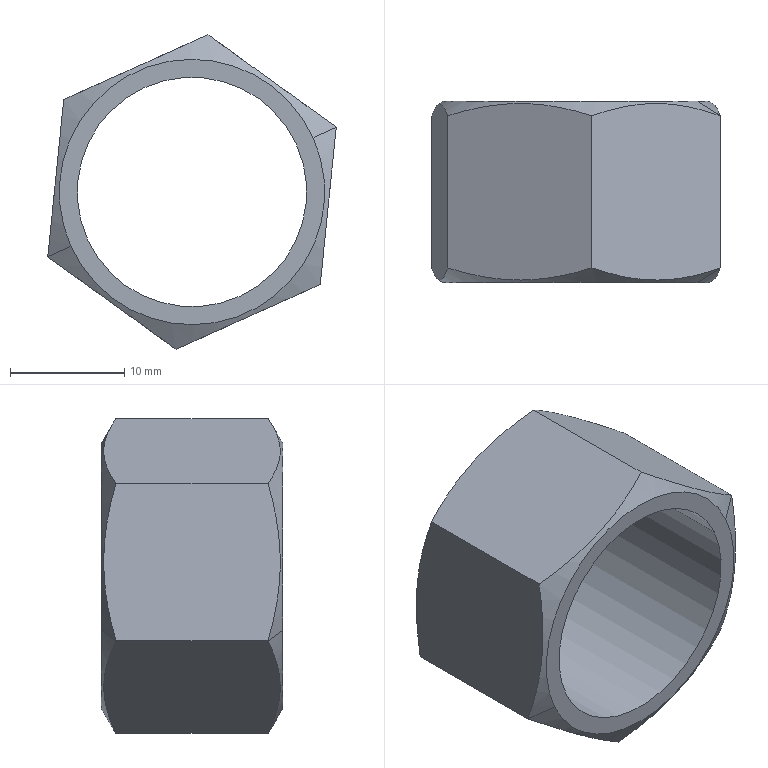Component | SolidWorks | YC1-250-04BalancerAssembly#16673-1_GBHexNutM20_GB_FASTENER_NUT_SNC1M16-N-1 | 1 solid | 14 faces | box 25.28 x 15.9 x 27.57 mm | volume 2830 mm3 | plane 8 | cone 4 | cylinder 2 | commonest cylinder face diameters 20.1 x2 | material Plain Carbon Steel
STEP:
#1=CARTESIAN_POINT('',(-13.739,185.201,-4.895));
#2=VERTEX_POINT('',#1);
#3=CARTESIAN_POINT('',(-13.017,185.201,-4.57));
#4=VERTEX_POINT('',#3);
#5=CARTESIAN_POINT('',(-13.378,185.201,-4.733));
#6=DIRECTION('',(-0.,1.,0.));
#7=DIRECTION('',(-0.9121,0.,-0.41));
#8=AXIS2_PLACEMENT_3D('',#5,#6,#7);
#9=CIRCLE('',#8,0.3957);
#10=EDGE_CURVE('',#2,#4,#9,.T.);
#11=ORIENTED_EDGE('',*,*,#10,.F.);
#12=CARTESIAN_POINT('',(-13.739,185.827,-4.895));
#13=VERTEX_POINT('',#12);
#14=CARTESIAN_POINT('',(-13.739,185.201,-4.895));
#15=DIRECTION('',(-0.,1.,0.));
#16=VECTOR('',#15,39.37);
#17=LINE('',#14,#16);
#18=EDGE_CURVE('',#2,#13,#17,.T.);
#19=ORIENTED_EDGE('',*,*,#18,.T.);
#20=CARTESIAN_POINT('',(-13.017,185.827,-4.57));
#21=VERTEX_POINT('',#20);
#22=CARTESIAN_POINT('',(-13.378,185.827,-4.733));
#23=DIRECTION('',(-0.,1.,0.));
#24=DIRECTION('',(-0.9121,0.,-0.41));
#25=AXIS2_PLACEMENT_3D('',#22,#23,#24);
#26=CIRCLE('',#25,0.3957);
#27=EDGE_CURVE('',#13,#21,#26,.T.);
#28=ORIENTED_EDGE('',*,*,#27,.T.);
#29=CARTESIAN_POINT('',(-13.017,185.201,-4.57));
#30=DIRECTION('',(-0.,1.,0.));
#31=VECTOR('',#30,39.37);
#32=LINE('',#29,#31);
#33=EDGE_CURVE('',#4,#21,#32,.T.);
#34=ORIENTED_EDGE('',*,*,#33,.F.);
#35=EDGE_LOOP('',(#11,#19,#28,#34));
#36=FACE_OUTER_BOUND('',#35,.T.);
#37=CARTESIAN_POINT('',(-13.378,185.201,-4.733));
#38=DIRECTION('',(-0.,1.,0.));
#39=DIRECTION('',(0.9121,0.,0.41));
#40=AXIS2_PLACEMENT_3D('',#37,#38,#39);
#41=CYLINDRICAL_SURFACE('',#40,0.3957);
#42=ADVANCED_FACE('',(#36),#41,.F.);
#43=CARTESIAN_POINT('',(-13.795,185.827,-4.92));
#44=VERTEX_POINT('',#43);
#45=CARTESIAN_POINT('',(-12.96,185.827,-4.545));
#46=VERTEX_POINT('',#45);
#47=CARTESIAN_POINT('',(-13.378,185.827,-4.733));
#48=DIRECTION('',(0.,-1.,-0.));
#49=DIRECTION('',(-0.9121,0.,-0.41));
#50=AXIS2_PLACEMENT_3D('',#47,#48,#49);
#51=CIRCLE('',#50,0.4577);
#52=EDGE_CURVE('',#44,#46,#51,.T.);
#53=ORIENTED_EDGE('',*,*,#52,.T.);
#54=CARTESIAN_POINT('',(-12.88,185.776,-4.509));
#55=VERTEX_POINT('',#54);
#56=CARTESIAN_POINT('',(-12.88,185.776,-4.509));
#57=DIRECTION('',(0.7899,-0.5,0.3551));
#58=VECTOR('',#57,39.37);
#59=LINE('',#56,#58);
#60=EDGE_CURVE('',#46,#55,#59,.T.);
#61=ORIENTED_EDGE('',*,*,#60,.T.);
#62=CARTESIAN_POINT('',(-12.935,185.776,-5.052));
#63=VERTEX_POINT('',#62);
#64=CARTESIAN_POINT('',(-12.88,185.776,-4.509));
#65=CARTESIAN_POINT('',(-12.885,185.789,-4.553));
#66=CARTESIAN_POINT('',(-12.889,185.8,-4.598));
#67=CARTESIAN_POINT('',(-12.898,185.814,-4.688));
#68=CARTESIAN_POINT('',(-12.903,185.818,-4.734));
#69=CARTESIAN_POINT('',(-12.91,185.818,-4.803));
#70=CARTESIAN_POINT('',(-12.912,185.817,-4.826));
#71=CARTESIAN_POINT('',(-12.917,185.813,-4.872));
#72=CARTESIAN_POINT('',(-12.919,185.811,-4.895));
#73=CARTESIAN_POINT('',(-12.926,185.8,-4.963));
#74=CARTESIAN_POINT('',(-12.931,185.789,-5.007));
#75=CARTESIAN_POINT('',(-12.935,185.776,-5.052));
#76=B_SPLINE_CURVE_WITH_KNOTS('',3,(#64,#65,#66,#67,#68,#69,#70,#71,#72,#73,#74,#75),.UNSPECIFIED.,.F.,.F.,(4,2,2,2,2,4),(0.,0.003499,0.006997,0.008746,0.0105,0.01399),.UNSPECIFIED.);
#77=EDGE_CURVE('',#55,#63,#76,.T.);
#78=ORIENTED_EDGE('',*,*,#77,.T.);
#79=CARTESIAN_POINT('',(-13.433,185.776,-5.275));
#80=VERTEX_POINT('',#79);
#81=CARTESIAN_POINT('',(-12.935,185.776,-5.052));
#82=CARTESIAN_POINT('',(-12.976,185.789,-5.07));
#83=CARTESIAN_POINT('',(-13.017,185.8,-5.088));
#84=CARTESIAN_POINT('',(-13.099,185.814,-5.125));
#85=CARTESIAN_POINT('',(-13.141,185.818,-5.144));
#86=CARTESIAN_POINT('',(-13.205,185.818,-5.173));
#87=CARTESIAN_POINT('',(-13.226,185.817,-5.182));
#88=CARTESIAN_POINT('',(-13.268,185.813,-5.201));
#89=CARTESIAN_POINT('',(-13.289,185.811,-5.211));
#90=CARTESIAN_POINT('',(-13.351,185.8,-5.239));
#91=CARTESIAN_POINT('',(-13.392,185.789,-5.257));
#92=CARTESIAN_POINT('',(-13.433,185.776,-5.275));
#93=B_SPLINE_CURVE_WITH_KNOTS('',3,(#81,#82,#83,#84,#85,#86,#87,#88,#89,#90,#91,#92),.UNSPECIFIED.,.F.,.F.,(4,2,2,2,2,4),(0.,0.003499,0.006997,0.008746,0.0105,0.01399),.UNSPECIFIED.);
#94=EDGE_CURVE('',#63,#80,#93,.T.);
#95=ORIENTED_EDGE('',*,*,#94,.T.);
#96=CARTESIAN_POINT('',(-13.875,185.776,-4.956));
#97=VERTEX_POINT('',#96);
#98=CARTESIAN_POINT('',(-13.433,185.776,-5.275));
#99=CARTESIAN_POINT('',(-13.469,185.789,-5.249));
#100=CARTESIAN_POINT('',(-13.505,185.8,-5.223));
#101=CARTESIAN_POINT('',(-13.579,185.814,-5.17));
#102=CARTESIAN_POINT('',(-13.616,185.818,-5.143));
#103=CARTESIAN_POINT('',(-13.672,185.818,-5.103));
#104=CARTESIAN_POINT('',(-13.691,185.817,-5.089));
#105=CARTESIAN_POINT('',(-13.729,185.813,-5.062));
#106=CARTESIAN_POINT('',(-13.747,185.811,-5.049));
#107=CARTESIAN_POINT('',(-13.803,185.8,-5.009));
#108=CARTESIAN_POINT('',(-13.839,185.789,-4.982));
#109=CARTESIAN_POINT('',(-13.875,185.776,-4.956));
#110=B_SPLINE_CURVE_WITH_KNOTS('',3,(#98,#99,#100,#101,#102,#103,#104,#105,#106,#107,#108,#109),.UNSPECIFIED.,.F.,.F.,(4,2,2,2,2,4),(0.,0.003499,0.006997,0.008746,0.0105,0.01399),.UNSPECIFIED.);
#111=EDGE_CURVE('',#80,#97,#110,.T.);
#112=ORIENTED_EDGE('',*,*,#111,.T.);
#113=CARTESIAN_POINT('',(-13.876,185.776,-4.957));
#114=DIRECTION('',(-0.7899,-0.5,-0.3551));
#115=VECTOR('',#114,39.37);
#116=LINE('',#113,#115);
#117=EDGE_CURVE('',#44,#97,#116,.T.);
#118=ORIENTED_EDGE('',*,*,#117,.F.);
#119=EDGE_LOOP('',(#53,#61,#78,#95,#112,#118));
#120=FACE_OUTER_BOUND('',#119,.T.);
#121=CARTESIAN_POINT('',(-13.378,185.776,-4.733));
#122=DIRECTION('',(0.,-1.,-0.));
#123=DIRECTION('',(-0.9121,0.,-0.41));
#124=AXIS2_PLACEMENT_3D('',#121,#122,#123);
#125=CONICAL_SURFACE('',#124,0.5461,1.047);
#126=ADVANCED_FACE('',(#120),#125,.T.);
#127=CARTESIAN_POINT('',(-13.795,185.201,-4.92));
#128=VERTEX_POINT('',#127);
#129=CARTESIAN_POINT('',(-12.96,185.201,-4.545));
#130=VERTEX_POINT('',#129);
#131=CARTESIAN_POINT('',(-13.378,185.201,-4.733));
#132=DIRECTION('',(0.,-1.,-0.));
#133=DIRECTION('',(0.9121,0.,0.41));
#134=AXIS2_PLACEMENT_3D('',#131,#132,#133);
#135=CIRCLE('',#134,0.4577);
#136=EDGE_CURVE('',#128,#130,#135,.T.);
#137=ORIENTED_EDGE('',*,*,#136,.F.);
#138=CARTESIAN_POINT('',(-13.875,185.252,-4.956));
#139=VERTEX_POINT('',#138);
#140=CARTESIAN_POINT('',(-13.876,185.252,-4.957));
#141=DIRECTION('',(-0.7899,0.5,-0.3551));
#142=VECTOR('',#141,39.37);
#143=LINE('',#140,#142);
#144=EDGE_CURVE('',#128,#139,#143,.T.);
#145=ORIENTED_EDGE('',*,*,#144,.T.);
#146=CARTESIAN_POINT('',(-13.433,185.252,-5.275));
#147=VERTEX_POINT('',#146);
#148=CARTESIAN_POINT('',(-13.875,185.252,-4.956));
#149=CARTESIAN_POINT('',(-13.839,185.239,-4.982));
#150=CARTESIAN_POINT('',(-13.803,185.228,-5.009));
#151=CARTESIAN_POINT('',(-13.729,185.213,-5.062));
#152=CARTESIAN_POINT('',(-13.692,185.209,-5.088));
#153=CARTESIAN_POINT('',(-13.636,185.209,-5.129));
#154=CARTESIAN_POINT('',(-13.617,185.21,-5.143));
#155=CARTESIAN_POINT('',(-13.579,185.214,-5.17));
#156=CARTESIAN_POINT('',(-13.561,185.217,-5.183));
#157=CARTESIAN_POINT('',(-13.505,185.228,-5.223));
#158=CARTESIAN_POINT('',(-13.469,185.239,-5.249));
#159=CARTESIAN_POINT('',(-13.433,185.252,-5.275));
#160=B_SPLINE_CURVE_WITH_KNOTS('',3,(#148,#149,#150,#151,#152,#153,#154,#155,#156,#157,#158,#159),.UNSPECIFIED.,.F.,.F.,(4,2,2,2,2,4),(0.,0.003499,0.006997,0.008746,0.0105,0.01399),.UNSPECIFIED.);
#161=EDGE_CURVE('',#139,#147,#160,.T.);
#162=ORIENTED_EDGE('',*,*,#161,.T.);
#163=CARTESIAN_POINT('',(-12.935,185.252,-5.052));
#164=VERTEX_POINT('',#163);
#165=CARTESIAN_POINT('',(-13.433,185.252,-5.275));
#166=CARTESIAN_POINT('',(-13.392,185.239,-5.257));
#167=CARTESIAN_POINT('',(-13.351,185.228,-5.239));
#168=CARTESIAN_POINT('',(-13.268,185.213,-5.202));
#169=CARTESIAN_POINT('',(-13.227,185.209,-5.183));
#170=CARTESIAN_POINT('',(-13.163,185.209,-5.154));
#171=CARTESIAN_POINT('',(-13.142,185.21,-5.145));
#172=CARTESIAN_POINT('',(-13.1,185.214,-5.126));
#173=CARTESIAN_POINT('',(-13.079,185.217,-5.116));
#174=CARTESIAN_POINT('',(-13.017,185.228,-5.088));
#175=CARTESIAN_POINT('',(-12.976,185.239,-5.07));
#176=CARTESIAN_POINT('',(-12.935,185.252,-5.052));
#177=B_SPLINE_CURVE_WITH_KNOTS('',3,(#165,#166,#167,#168,#169,#170,#171,#172,#173,#174,#175,#176),.UNSPECIFIED.,.F.,.F.,(4,2,2,2,2,4),(0.,0.003499,0.006997,0.008746,0.0105,0.01399),.UNSPECIFIED.);
#178=EDGE_CURVE('',#147,#164,#177,.T.);
#179=ORIENTED_EDGE('',*,*,#178,.T.);
#180=CARTESIAN_POINT('',(-12.88,185.252,-4.509));
#181=VERTEX_POINT('',#180);
#182=CARTESIAN_POINT('',(-12.935,185.252,-5.052));
#183=CARTESIAN_POINT('',(-12.931,185.239,-5.007));
#184=CARTESIAN_POINT('',(-12.926,185.228,-4.963));
#185=CARTESIAN_POINT('',(-12.917,185.213,-4.873));
#186=CARTESIAN_POINT('',(-12.912,185.209,-4.827));
#187=CARTESIAN_POINT('',(-12.905,185.209,-4.758));
#188=CARTESIAN_POINT('',(-12.903,185.21,-4.735));
#189=CARTESIAN_POINT('',(-12.898,185.214,-4.689));
#190=CARTESIAN_POINT('',(-12.896,185.217,-4.666));
#191=CARTESIAN_POINT('',(-12.889,185.228,-4.598));
#192=CARTESIAN_POINT('',(-12.885,185.239,-4.553));
#193=CARTESIAN_POINT('',(-12.88,185.252,-4.509));
#194=B_SPLINE_CURVE_WITH_KNOTS('',3,(#182,#183,#184,#185,#186,#187,#188,#189,#190,#191,#192,#193),.UNSPECIFIED.,.F.,.F.,(4,2,2,2,2,4),(0.,0.003499,0.006997,0.008746,0.0105,0.01399),.UNSPECIFIED.);
#195=EDGE_CURVE('',#164,#181,#194,.T.);
#196=ORIENTED_EDGE('',*,*,#195,.T.);
#197=CARTESIAN_POINT('',(-12.88,185.252,-4.509));
#198=DIRECTION('',(0.7899,0.5,0.3551));
#199=VECTOR('',#198,39.37);
#200=LINE('',#197,#199);
#201=EDGE_CURVE('',#130,#181,#200,.T.);
#202=ORIENTED_EDGE('',*,*,#201,.F.);
#203=EDGE_LOOP('',(#137,#145,#162,#179,#196,#202));
#204=FACE_OUTER_BOUND('',#203,.T.);
#205=CARTESIAN_POINT('',(-13.378,185.252,-4.733));
#206=DIRECTION('',(-0.,1.,0.));
#207=DIRECTION('',(0.9121,0.,0.41));
#208=AXIS2_PLACEMENT_3D('',#205,#206,#207);
#209=CONICAL_SURFACE('',#208,0.5461,1.047);
#210=ADVANCED_FACE('',(#204),#209,.T.);
#211=CARTESIAN_POINT('',(-13.378,185.827,-4.733));
#212=DIRECTION('',(-0.,1.,0.));
#213=DIRECTION('',(-0.9121,0.,-0.41));
#214=AXIS2_PLACEMENT_3D('',#211,#212,#213);
#215=CIRCLE('',#214,0.3957);
#216=EDGE_CURVE('',#21,#13,#215,.T.);
#217=ORIENTED_EDGE('',*,*,#216,.F.);
#218=ORIENTED_EDGE('',*,*,#27,.F.);
#219=EDGE_LOOP('',(#217,#218));
#220=FACE_BOUND('',#219,.T.);
#221=ORIENTED_EDGE('',*,*,#52,.F.);
#222=CARTESIAN_POINT('',(-13.378,185.827,-4.733));
#223=DIRECTION('',(0.,-1.,-0.));
#224=DIRECTION('',(-0.9121,0.,-0.41));
#225=AXIS2_PLACEMENT_3D('',#222,#223,#224);
#226=CIRCLE('',#225,0.4577);
#227=EDGE_CURVE('',#46,#44,#226,.T.);
#228=ORIENTED_EDGE('',*,*,#227,.F.);
#229=EDGE_LOOP('',(#221,#228));
#230=FACE_OUTER_BOUND('',#229,.T.);
#231=CARTESIAN_POINT('',(-13.82,185.827,-4.414));
#232=DIRECTION('',(0.,-1.,-0.));
#233=DIRECTION('',(-0.9121,0.,-0.41));
#234=AXIS2_PLACEMENT_3D('',#231,#232,#233);
#235=PLANE('',#234);
#236=ADVANCED_FACE('',(#220,#230),#235,.F.);
#237=CARTESIAN_POINT('',(-13.378,185.201,-4.733));
#238=DIRECTION('',(-0.,1.,0.));
#239=DIRECTION('',(-0.9121,0.,-0.41));
#240=AXIS2_PLACEMENT_3D('',#237,#238,#239);
#241=CIRCLE('',#240,0.3957);
#242=EDGE_CURVE('',#4,#2,#241,.T.);
#243=ORIENTED_EDGE('',*,*,#242,.T.);
#244=ORIENTED_EDGE('',*,*,#10,.T.);
#245=EDGE_LOOP('',(#243,#244));
#246=FACE_BOUND('',#245,.T.);
#247=CARTESIAN_POINT('',(-13.378,185.201,-4.733));
#248=DIRECTION('',(0.,-1.,-0.));
#249=DIRECTION('',(0.9121,0.,0.41));
#250=AXIS2_PLACEMENT_3D('',#247,#248,#249);
#251=CIRCLE('',#250,0.4577);
#252=EDGE_CURVE('',#130,#128,#251,.T.);
#253=ORIENTED_EDGE('',*,*,#252,.T.);
#254=ORIENTED_EDGE('',*,*,#136,.T.);
#255=EDGE_LOOP('',(#253,#254));
#256=FACE_OUTER_BOUND('',#255,.T.);
#257=CARTESIAN_POINT('',(-13.82,185.201,-4.414));
#258=DIRECTION('',(0.,-1.,-0.));
#259=DIRECTION('',(-0.9121,0.,-0.41));
#260=AXIS2_PLACEMENT_3D('',#257,#258,#259);
#261=PLANE('',#260);
#262=ADVANCED_FACE('',(#246,#256),#261,.T.);
#263=ORIENTED_EDGE('',*,*,#60,.F.);
#264=ORIENTED_EDGE('',*,*,#227,.T.);
#265=ORIENTED_EDGE('',*,*,#117,.T.);
#266=CARTESIAN_POINT('',(-13.82,185.776,-4.414));
#267=VERTEX_POINT('',#266);
#268=CARTESIAN_POINT('',(-13.875,185.776,-4.956));
#269=CARTESIAN_POINT('',(-13.871,185.789,-4.912));
#270=CARTESIAN_POINT('',(-13.866,185.8,-4.867));
#271=CARTESIAN_POINT('',(-13.857,185.814,-4.777));
#272=CARTESIAN_POINT('',(-13.852,185.818,-4.732));
#273=CARTESIAN_POINT('',(-13.845,185.818,-4.662));
#274=CARTESIAN_POINT('',(-13.843,185.817,-4.639));
#275=CARTESIAN_POINT('',(-13.838,185.813,-4.593));
#276=CARTESIAN_POINT('',(-13.836,185.811,-4.571));
#277=CARTESIAN_POINT('',(-13.829,185.8,-4.503));
#278=CARTESIAN_POINT('',(-13.825,185.789,-4.458));
#279=CARTESIAN_POINT('',(-13.82,185.776,-4.414));
#280=B_SPLINE_CURVE_WITH_KNOTS('',3,(#268,#269,#270,#271,#272,#273,#274,#275,#276,#277,#278,#279),.UNSPECIFIED.,.F.,.F.,(4,2,2,2,2,4),(0.,0.003499,0.006997,0.008746,0.0105,0.01399),.UNSPECIFIED.);
#281=EDGE_CURVE('',#97,#267,#280,.T.);
#282=ORIENTED_EDGE('',*,*,#281,.T.);
#283=CARTESIAN_POINT('',(-13.323,185.776,-4.19));
#284=VERTEX_POINT('',#283);
#285=CARTESIAN_POINT('',(-13.82,185.776,-4.414));
#286=CARTESIAN_POINT('',(-13.78,185.789,-4.395));
#287=CARTESIAN_POINT('',(-13.739,185.8,-4.377));
#288=CARTESIAN_POINT('',(-13.656,185.814,-4.34));
#289=CARTESIAN_POINT('',(-13.614,185.818,-4.321));
#290=CARTESIAN_POINT('',(-13.551,185.818,-4.292));
#291=CARTESIAN_POINT('',(-13.529,185.817,-4.283));
#292=CARTESIAN_POINT('',(-13.487,185.813,-4.264));
#293=CARTESIAN_POINT('',(-13.467,185.811,-4.255));
#294=CARTESIAN_POINT('',(-13.404,185.8,-4.227));
#295=CARTESIAN_POINT('',(-13.363,185.789,-4.208));
#296=CARTESIAN_POINT('',(-13.323,185.776,-4.19));
#297=B_SPLINE_CURVE_WITH_KNOTS('',3,(#285,#286,#287,#288,#289,#290,#291,#292,#293,#294,#295,#296),.UNSPECIFIED.,.F.,.F.,(4,2,2,2,2,4),(0.,0.003499,0.006997,0.008746,0.0105,0.01399),.UNSPECIFIED.);
#298=EDGE_CURVE('',#267,#284,#297,.T.);
#299=ORIENTED_EDGE('',*,*,#298,.T.);
#300=CARTESIAN_POINT('',(-13.323,185.776,-4.19));
#301=CARTESIAN_POINT('',(-13.286,185.789,-4.216));
#302=CARTESIAN_POINT('',(-13.25,185.8,-4.242));
#303=CARTESIAN_POINT('',(-13.177,185.814,-4.295));
#304=CARTESIAN_POINT('',(-13.139,185.818,-4.322));
#305=CARTESIAN_POINT('',(-13.083,185.818,-4.363));
#306=CARTESIAN_POINT('',(-13.064,185.817,-4.376));
#307=CARTESIAN_POINT('',(-13.027,185.813,-4.403));
#308=CARTESIAN_POINT('',(-13.008,185.811,-4.417));
#309=CARTESIAN_POINT('',(-12.953,185.8,-4.457));
#310=CARTESIAN_POINT('',(-12.916,185.789,-4.483));
#311=CARTESIAN_POINT('',(-12.88,185.776,-4.509));
#312=B_SPLINE_CURVE_WITH_KNOTS('',3,(#300,#301,#302,#303,#304,#305,#306,#307,#308,#309,#310,#311),.UNSPECIFIED.,.F.,.F.,(4,2,2,2,2,4),(0.,0.003499,0.006997,0.008746,0.0105,0.01399),.UNSPECIFIED.);
#313=EDGE_CURVE('',#284,#55,#312,.T.);
#314=ORIENTED_EDGE('',*,*,#313,.T.);
#315=EDGE_LOOP('',(#263,#264,#265,#282,#299,#314));
#316=FACE_OUTER_BOUND('',#315,.T.);
#317=CARTESIAN_POINT('',(-13.378,185.776,-4.733));
#318=DIRECTION('',(0.,-1.,-0.));
#319=DIRECTION('',(-0.9121,0.,-0.41));
#320=AXIS2_PLACEMENT_3D('',#317,#318,#319);
#321=CONICAL_SURFACE('',#320,0.5461,1.047);
#322=ADVANCED_FACE('',(#316),#321,.T.);
#323=ORIENTED_EDGE('',*,*,#144,.F.);
#324=ORIENTED_EDGE('',*,*,#252,.F.);
#325=ORIENTED_EDGE('',*,*,#201,.T.);
#326=CARTESIAN_POINT('',(-13.323,185.252,-4.19));
#327=VERTEX_POINT('',#326);
#328=CARTESIAN_POINT('',(-12.88,185.252,-4.509));
#329=CARTESIAN_POINT('',(-12.916,185.239,-4.483));
#330=CARTESIAN_POINT('',(-12.953,185.228,-4.457));
#331=CARTESIAN_POINT('',(-13.026,185.213,-4.404));
#332=CARTESIAN_POINT('',(-13.063,185.209,-4.377));
#333=CARTESIAN_POINT('',(-13.12,185.209,-4.336));
#334=CARTESIAN_POINT('',(-13.139,185.21,-4.323));
#335=CARTESIAN_POINT('',(-13.176,185.214,-4.296));
#336=CARTESIAN_POINT('',(-13.195,185.217,-4.282));
#337=CARTESIAN_POINT('',(-13.25,185.228,-4.242));
#338=CARTESIAN_POINT('',(-13.286,185.239,-4.216));
#339=CARTESIAN_POINT('',(-13.323,185.252,-4.19));
#340=B_SPLINE_CURVE_WITH_KNOTS('',3,(#328,#329,#330,#331,#332,#333,#334,#335,#336,#337,#338,#339),.UNSPECIFIED.,.F.,.F.,(4,2,2,2,2,4),(0.,0.003499,0.006997,0.008746,0.0105,0.01399),.UNSPECIFIED.);
#341=EDGE_CURVE('',#181,#327,#340,.T.);
#342=ORIENTED_EDGE('',*,*,#341,.T.);
#343=CARTESIAN_POINT('',(-13.82,185.252,-4.414));
#344=VERTEX_POINT('',#343);
#345=CARTESIAN_POINT('',(-13.323,185.252,-4.19));
#346=CARTESIAN_POINT('',(-13.363,185.239,-4.208));
#347=CARTESIAN_POINT('',(-13.404,185.228,-4.227));
#348=CARTESIAN_POINT('',(-13.487,185.213,-4.264));
#349=CARTESIAN_POINT('',(-13.529,185.209,-4.282));
#350=CARTESIAN_POINT('',(-13.592,185.209,-4.311));
#351=CARTESIAN_POINT('',(-13.613,185.21,-4.321));
#352=CARTESIAN_POINT('',(-13.655,185.214,-4.339));
#353=CARTESIAN_POINT('',(-13.676,185.217,-4.349));
#354=CARTESIAN_POINT('',(-13.738,185.228,-4.377));
#355=CARTESIAN_POINT('',(-13.779,185.239,-4.395));
#356=CARTESIAN_POINT('',(-13.82,185.252,-4.414));
#357=B_SPLINE_CURVE_WITH_KNOTS('',3,(#345,#346,#347,#348,#349,#350,#351,#352,#353,#354,#355,#356),.UNSPECIFIED.,.F.,.F.,(4,2,2,2,2,4),(0.,0.003499,0.006997,0.008746,0.0105,0.01399),.UNSPECIFIED.);
#358=EDGE_CURVE('',#327,#344,#357,.T.);
#359=ORIENTED_EDGE('',*,*,#358,.T.);
#360=CARTESIAN_POINT('',(-13.82,185.252,-4.414));
#361=CARTESIAN_POINT('',(-13.825,185.239,-4.458));
#362=CARTESIAN_POINT('',(-13.829,185.228,-4.502));
#363=CARTESIAN_POINT('',(-13.838,185.213,-4.593));
#364=CARTESIAN_POINT('',(-13.843,185.209,-4.638));
#365=CARTESIAN_POINT('',(-13.85,185.209,-4.707));
#366=CARTESIAN_POINT('',(-13.852,185.21,-4.731));
#367=CARTESIAN_POINT('',(-13.857,185.214,-4.777));
#368=CARTESIAN_POINT('',(-13.859,185.217,-4.799));
#369=CARTESIAN_POINT('',(-13.866,185.228,-4.867));
#370=CARTESIAN_POINT('',(-13.871,185.239,-4.912));
#371=CARTESIAN_POINT('',(-13.875,185.252,-4.956));
#372=B_SPLINE_CURVE_WITH_KNOTS('',3,(#360,#361,#362,#363,#364,#365,#366,#367,#368,#369,#370,#371),.UNSPECIFIED.,.F.,.F.,(4,2,2,2,2,4),(0.,0.003499,0.006997,0.008746,0.0105,0.01399),.UNSPECIFIED.);
#373=EDGE_CURVE('',#344,#139,#372,.T.);
#374=ORIENTED_EDGE('',*,*,#373,.T.);
#375=EDGE_LOOP('',(#323,#324,#325,#342,#359,#374));
#376=FACE_OUTER_BOUND('',#375,.T.);
#377=CARTESIAN_POINT('',(-13.378,185.252,-4.733));
#378=DIRECTION('',(-0.,1.,0.));
#379=DIRECTION('',(0.9121,0.,0.41));
#380=AXIS2_PLACEMENT_3D('',#377,#378,#379);
#381=CONICAL_SURFACE('',#380,0.5461,1.047);
#382=ADVANCED_FACE('',(#376),#381,.T.);
#383=ORIENTED_EDGE('',*,*,#313,.F.);
#384=CARTESIAN_POINT('',(-13.323,185.827,-4.19));
#385=DIRECTION('',(0.,-1.,-0.));
#386=VECTOR('',#385,39.37);
#387=LINE('',#384,#386);
#388=EDGE_CURVE('',#284,#327,#387,.T.);
#389=ORIENTED_EDGE('',*,*,#388,.T.);
#390=ORIENTED_EDGE('',*,*,#341,.F.);
#391=CARTESIAN_POINT('',(-12.88,185.827,-4.509));
#392=DIRECTION('',(-0.,1.,0.));
#393=VECTOR('',#392,39.37);
#394=LINE('',#391,#393);
#395=EDGE_CURVE('',#181,#55,#394,.T.);
#396=ORIENTED_EDGE('',*,*,#395,.T.);
#397=EDGE_LOOP('',(#383,#389,#390,#396));
#398=FACE_OUTER_BOUND('',#397,.T.);
#399=CARTESIAN_POINT('',(-12.88,185.827,-4.509));
#400=DIRECTION('',(0.5848,-0.,0.8111));
#401=DIRECTION('',(-0.8111,-0.,0.5848));
#402=AXIS2_PLACEMENT_3D('',#399,#400,#401);
#403=PLANE('',#402);
#404=ADVANCED_FACE('',(#398),#403,.T.);
#405=ORIENTED_EDGE('',*,*,#298,.F.);
#406=CARTESIAN_POINT('',(-13.82,185.827,-4.414));
#407=DIRECTION('',(0.,-1.,-0.));
#408=VECTOR('',#407,39.37);
#409=LINE('',#406,#408);
#410=EDGE_CURVE('',#267,#344,#409,.T.);
#411=ORIENTED_EDGE('',*,*,#410,.T.);
#412=ORIENTED_EDGE('',*,*,#358,.F.);
#413=ORIENTED_EDGE('',*,*,#388,.F.);
#414=EDGE_LOOP('',(#405,#411,#412,#413));
#415=FACE_OUTER_BOUND('',#414,.T.);
#416=CARTESIAN_POINT('',(-13.323,185.827,-4.19));
#417=DIRECTION('',(-0.41,-0.,0.9121));
#418=DIRECTION('',(-0.9121,0.,-0.41));
#419=AXIS2_PLACEMENT_3D('',#416,#417,#418);
#420=PLANE('',#419);
#421=ADVANCED_FACE('',(#415),#420,.T.);
#422=ORIENTED_EDGE('',*,*,#281,.F.);
#423=CARTESIAN_POINT('',(-13.875,185.827,-4.956));
#424=DIRECTION('',(0.,-1.,-0.));
#425=VECTOR('',#424,39.37);
#426=LINE('',#423,#425);
#427=EDGE_CURVE('',#97,#139,#426,.T.);
#428=ORIENTED_EDGE('',*,*,#427,.T.);
#429=ORIENTED_EDGE('',*,*,#373,.F.);
#430=ORIENTED_EDGE('',*,*,#410,.F.);
#431=EDGE_LOOP('',(#422,#428,#429,#430));
#432=FACE_OUTER_BOUND('',#431,.T.);
#433=CARTESIAN_POINT('',(-13.82,185.827,-4.414));
#434=DIRECTION('',(-0.9949,-0.,0.1009));
#435=DIRECTION('',(-0.1009,0.,-0.9949));
#436=AXIS2_PLACEMENT_3D('',#433,#434,#435);
#437=PLANE('',#436);
#438=ADVANCED_FACE('',(#432),#437,.T.);
#439=ORIENTED_EDGE('',*,*,#111,.F.);
#440=CARTESIAN_POINT('',(-13.433,185.827,-5.275));
#441=DIRECTION('',(0.,-1.,-0.));
#442=VECTOR('',#441,39.37);
#443=LINE('',#440,#442);
#444=EDGE_CURVE('',#80,#147,#443,.T.);
#445=ORIENTED_EDGE('',*,*,#444,.T.);
#446=ORIENTED_EDGE('',*,*,#161,.F.);
#447=ORIENTED_EDGE('',*,*,#427,.F.);
#448=EDGE_LOOP('',(#439,#445,#446,#447));
#449=FACE_OUTER_BOUND('',#448,.T.);
#450=CARTESIAN_POINT('',(-13.875,185.827,-4.956));
#451=DIRECTION('',(-0.5848,0.,-0.8111));
#452=DIRECTION('',(0.8111,0.,-0.5848));
#453=AXIS2_PLACEMENT_3D('',#450,#451,#452);
#454=PLANE('',#453);
#455=ADVANCED_FACE('',(#449),#454,.T.);
#456=ORIENTED_EDGE('',*,*,#94,.F.);
#457=CARTESIAN_POINT('',(-12.935,185.827,-5.052));
#458=DIRECTION('',(0.,-1.,-0.));
#459=VECTOR('',#458,39.37);
#460=LINE('',#457,#459);
#461=EDGE_CURVE('',#63,#164,#460,.T.);
#462=ORIENTED_EDGE('',*,*,#461,.T.);
#463=ORIENTED_EDGE('',*,*,#178,.F.);
#464=ORIENTED_EDGE('',*,*,#444,.F.);
#465=EDGE_LOOP('',(#456,#462,#463,#464));
#466=FACE_OUTER_BOUND('',#465,.T.);
#467=CARTESIAN_POINT('',(-13.433,185.827,-5.275));
#468=DIRECTION('',(0.41,0.,-0.9121));
#469=DIRECTION('',(0.,-1.,-0.));
#470=AXIS2_PLACEMENT_3D('',#467,#468,#469);
#471=PLANE('',#470);
#472=ADVANCED_FACE('',(#466),#471,.T.);
#473=ORIENTED_EDGE('',*,*,#77,.F.);
#474=ORIENTED_EDGE('',*,*,#395,.F.);
#475=ORIENTED_EDGE('',*,*,#195,.F.);
#476=ORIENTED_EDGE('',*,*,#461,.F.);
#477=EDGE_LOOP('',(#473,#474,#475,#476));
#478=FACE_OUTER_BOUND('',#477,.T.);
#479=CARTESIAN_POINT('',(-12.935,185.827,-5.052));
#480=DIRECTION('',(0.9949,0.,-0.1009));
#481=DIRECTION('',(0.1009,-0.,0.9949));
#482=AXIS2_PLACEMENT_3D('',#479,#480,#481);
#483=PLANE('',#482);
#484=ADVANCED_FACE('',(#478),#483,.T.);
#485=ORIENTED_EDGE('',*,*,#18,.F.);
#486=ORIENTED_EDGE('',*,*,#242,.F.);
#487=ORIENTED_EDGE('',*,*,#33,.T.);
#488=ORIENTED_EDGE('',*,*,#216,.T.);
#489=EDGE_LOOP('',(#485,#486,#487,#488));
#490=FACE_OUTER_BOUND('',#489,.T.);
#491=CARTESIAN_POINT('',(-13.378,185.201,-4.733));
#492=DIRECTION('',(-0.,1.,0.));
#493=DIRECTION('',(0.9121,0.,0.41));
#494=AXIS2_PLACEMENT_3D('',#491,#492,#493);
#495=CYLINDRICAL_SURFACE('',#494,0.3957);
#496=ADVANCED_FACE('',(#490),#495,.F.);
#497=CLOSED_SHELL('',(#42,#126,#210,#236,#262,#322,#382,#404,#421,#438,#455,#472,#484,#496));
#498=MANIFOLD_SOLID_BREP('',#497);
#499=CARTESIAN_POINT('',(0.,0.,0.));
#500=DIRECTION('',(0.,0.,1.));
#501=DIRECTION('',(1.,0.,0.));
#502=AXIS2_PLACEMENT_3D('',#499,#500,#501);
#503=(LENGTH_UNIT()NAMED_UNIT(*)SI_UNIT($,.METRE.));
#504=LENGTH_MEASURE_WITH_UNIT(LENGTH_MEASURE(0.0254),#503);
#505=DIMENSIONAL_EXPONENTS(1.,0.,0.,0.,0.,0.,0.);
#506=(CONVERSION_BASED_UNIT('',#504)LENGTH_UNIT()NAMED_UNIT(#505));
#507=UNCERTAINTY_MEASURE_WITH_UNIT(LENGTH_MEASURE(0.00001),#506,'','');
#508=(NAMED_UNIT(*)PLANE_ANGLE_UNIT()SI_UNIT($,.RADIAN.));
#509=(NAMED_UNIT(*)SI_UNIT($,.STERADIAN.)SOLID_ANGLE_UNIT());
#510=(GEOMETRIC_REPRESENTATION_CONTEXT(3)GLOBAL_UNCERTAINTY_ASSIGNED_CONTEXT((#507))GLOBAL_UNIT_ASSIGNED_CONTEXT((#506,#508,#509))REPRESENTATION_CONTEXT('',''));
#511=ADVANCED_BREP_SHAPE_REPRESENTATION('',(#498,#502),#510);
#512=COLOUR_RGB('',0.7922,0.8196,0.9333);
#513=FILL_AREA_STYLE_COLOUR('',#512);
#514=FILL_AREA_STYLE('',(#513));
#515=SURFACE_STYLE_FILL_AREA(#514);
#516=SURFACE_SIDE_STYLE('',(#515));
#517=SURFACE_STYLE_USAGE(.BOTH.,#516);
#518=PRESENTATION_STYLE_ASSIGNMENT((#517));
#519=STYLED_ITEM('',(#518),#498);
#520=(LENGTH_UNIT()NAMED_UNIT(*)SI_UNIT($,.METRE.));
#521=LENGTH_MEASURE_WITH_UNIT(LENGTH_MEASURE(0.0254),#520);
#522=DIMENSIONAL_EXPONENTS(1.,0.,0.,0.,0.,0.,0.);
#523=(CONVERSION_BASED_UNIT('',#521)LENGTH_UNIT()NAMED_UNIT(#522));
#524=UNCERTAINTY_MEASURE_WITH_UNIT(LENGTH_MEASURE(0.00001),#523,'','');
#525=(NAMED_UNIT(*)PLANE_ANGLE_UNIT()SI_UNIT($,.RADIAN.));
#526=(NAMED_UNIT(*)SI_UNIT($,.STERADIAN.)SOLID_ANGLE_UNIT());
#527=(GEOMETRIC_REPRESENTATION_CONTEXT(3)GLOBAL_UNCERTAINTY_ASSIGNED_CONTEXT((#524))GLOBAL_UNIT_ASSIGNED_CONTEXT((#523,#525,#526))REPRESENTATION_CONTEXT('',''));
#528=MECHANICAL_DESIGN_GEOMETRIC_PRESENTATION_REPRESENTATION('',(#519),#527);
#529=PRESENTATION_LAYER_ASSIGNMENT('','',(#519));